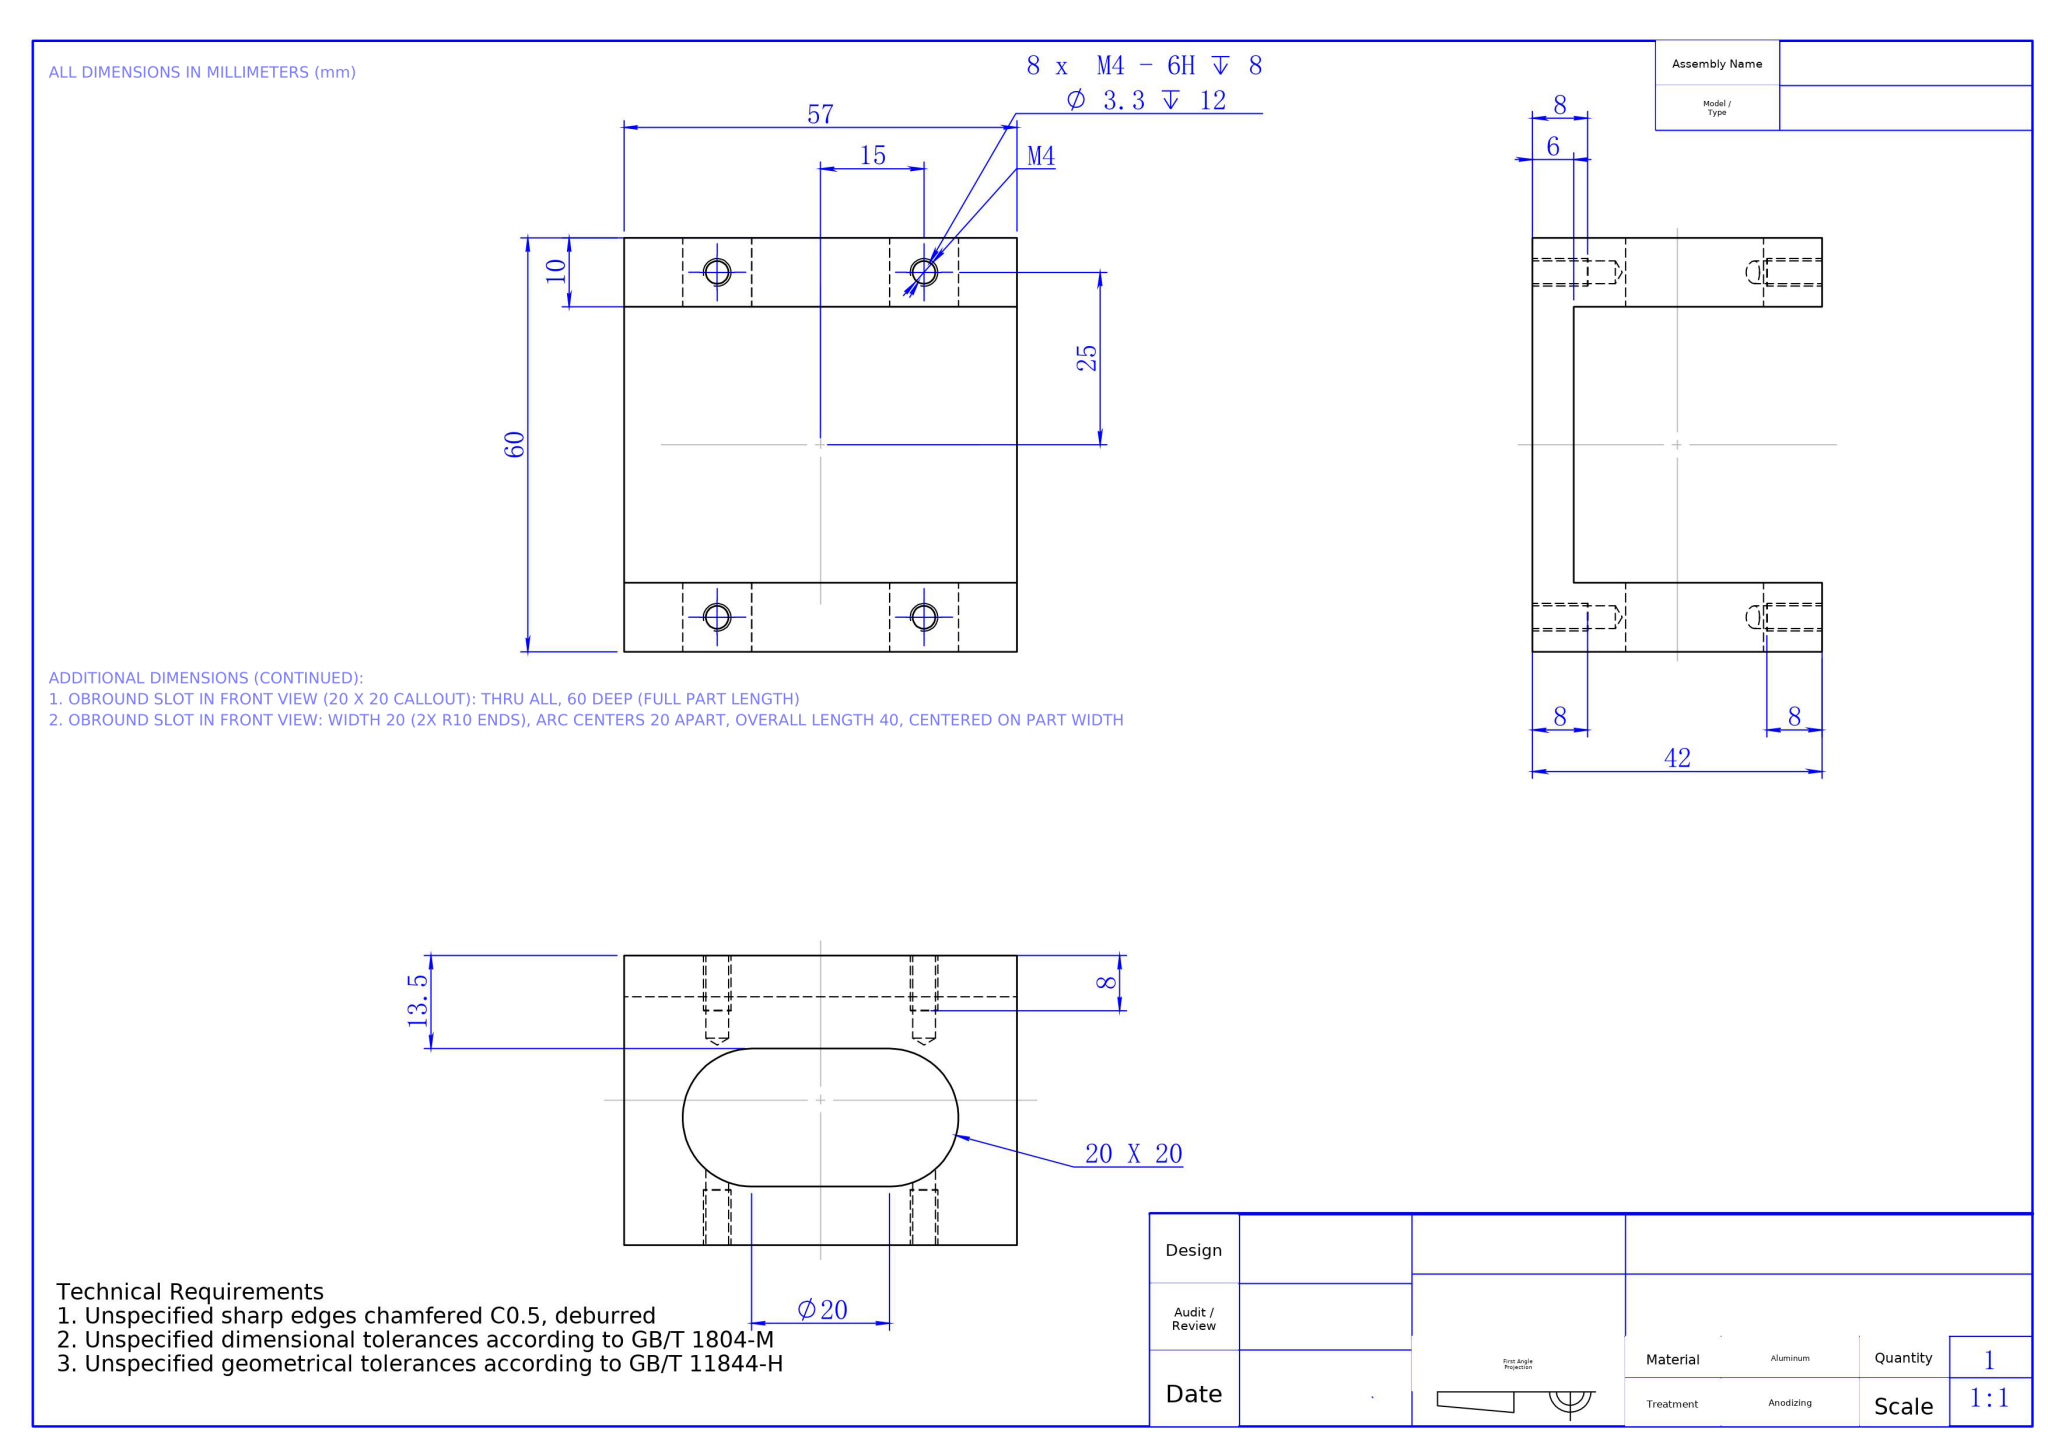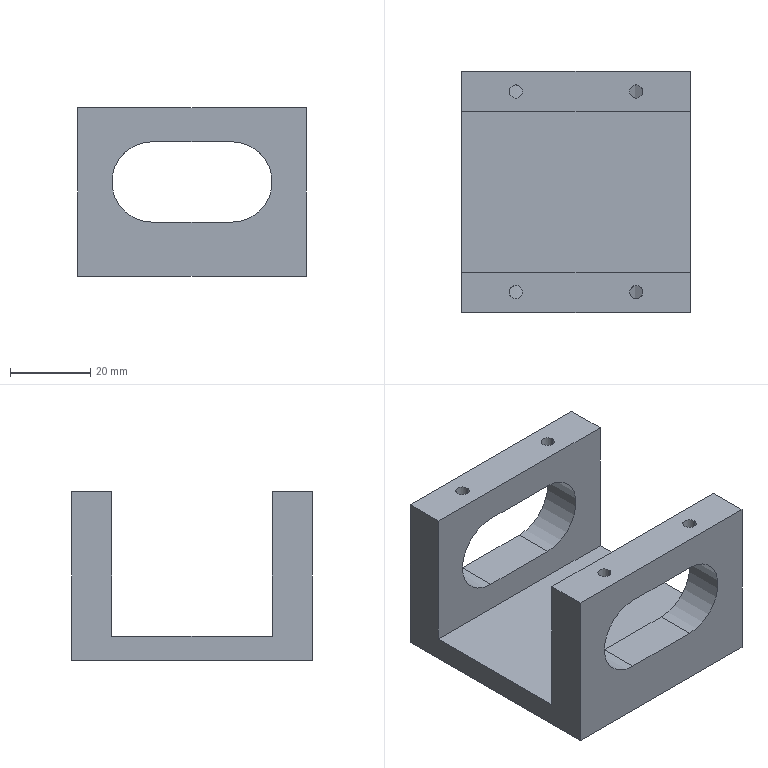Part | NX | mm | 1 solid | 42 faces | box 57 x 60 x 42 mm | volume 46517 mm3 | cylinder 20 | plane 14 | cone 8 | commonest cylinder face diameters 3.3 x16 20 x4